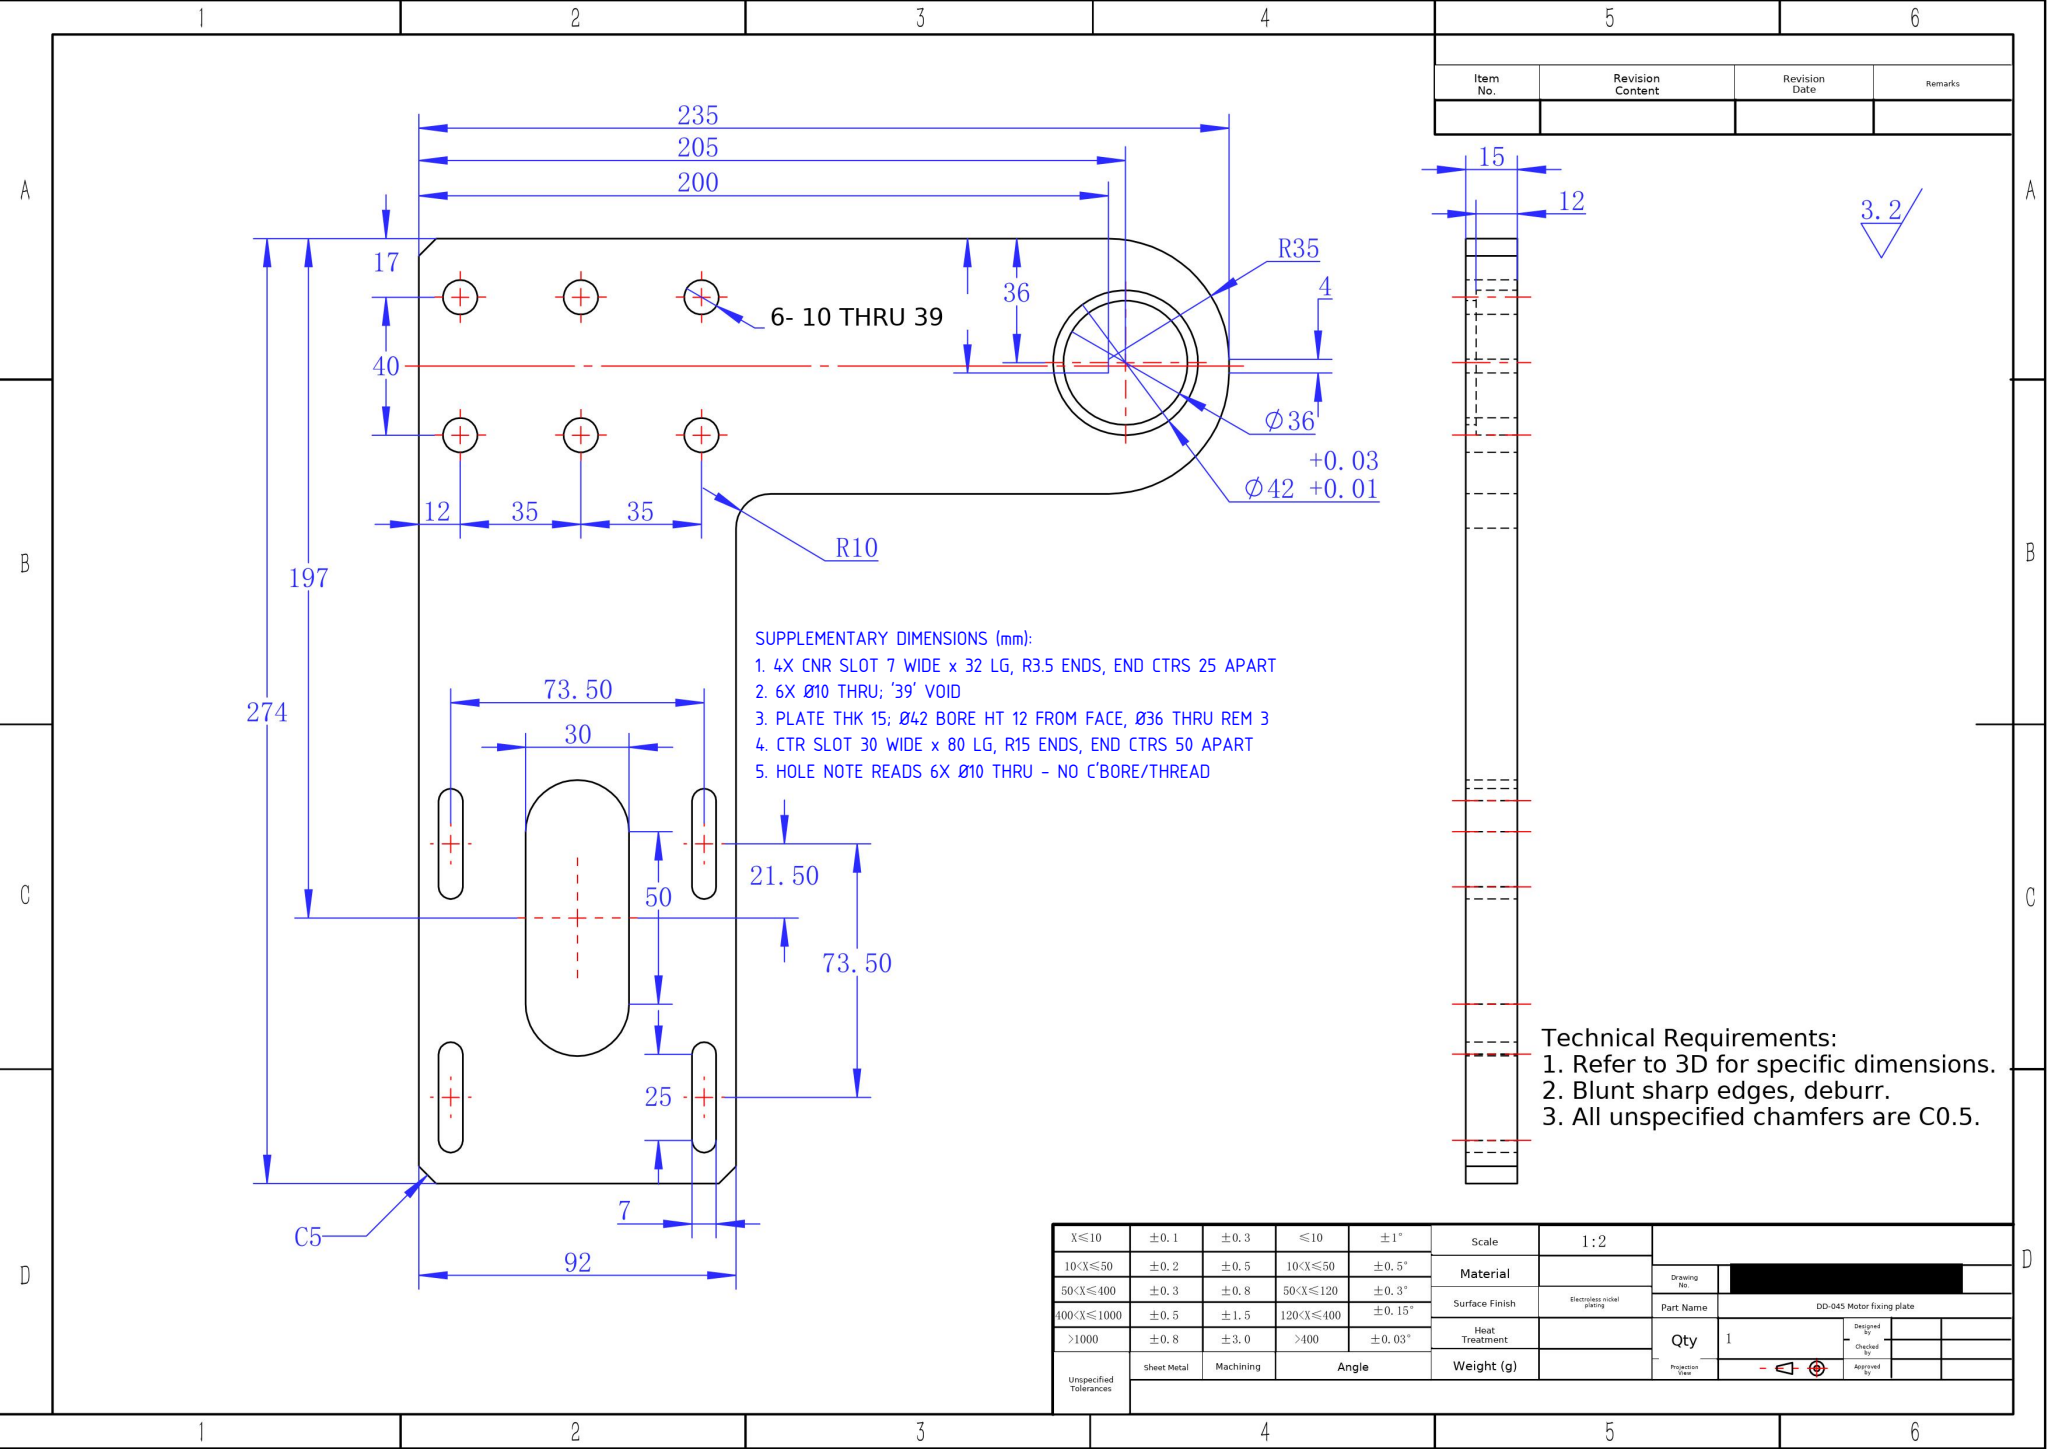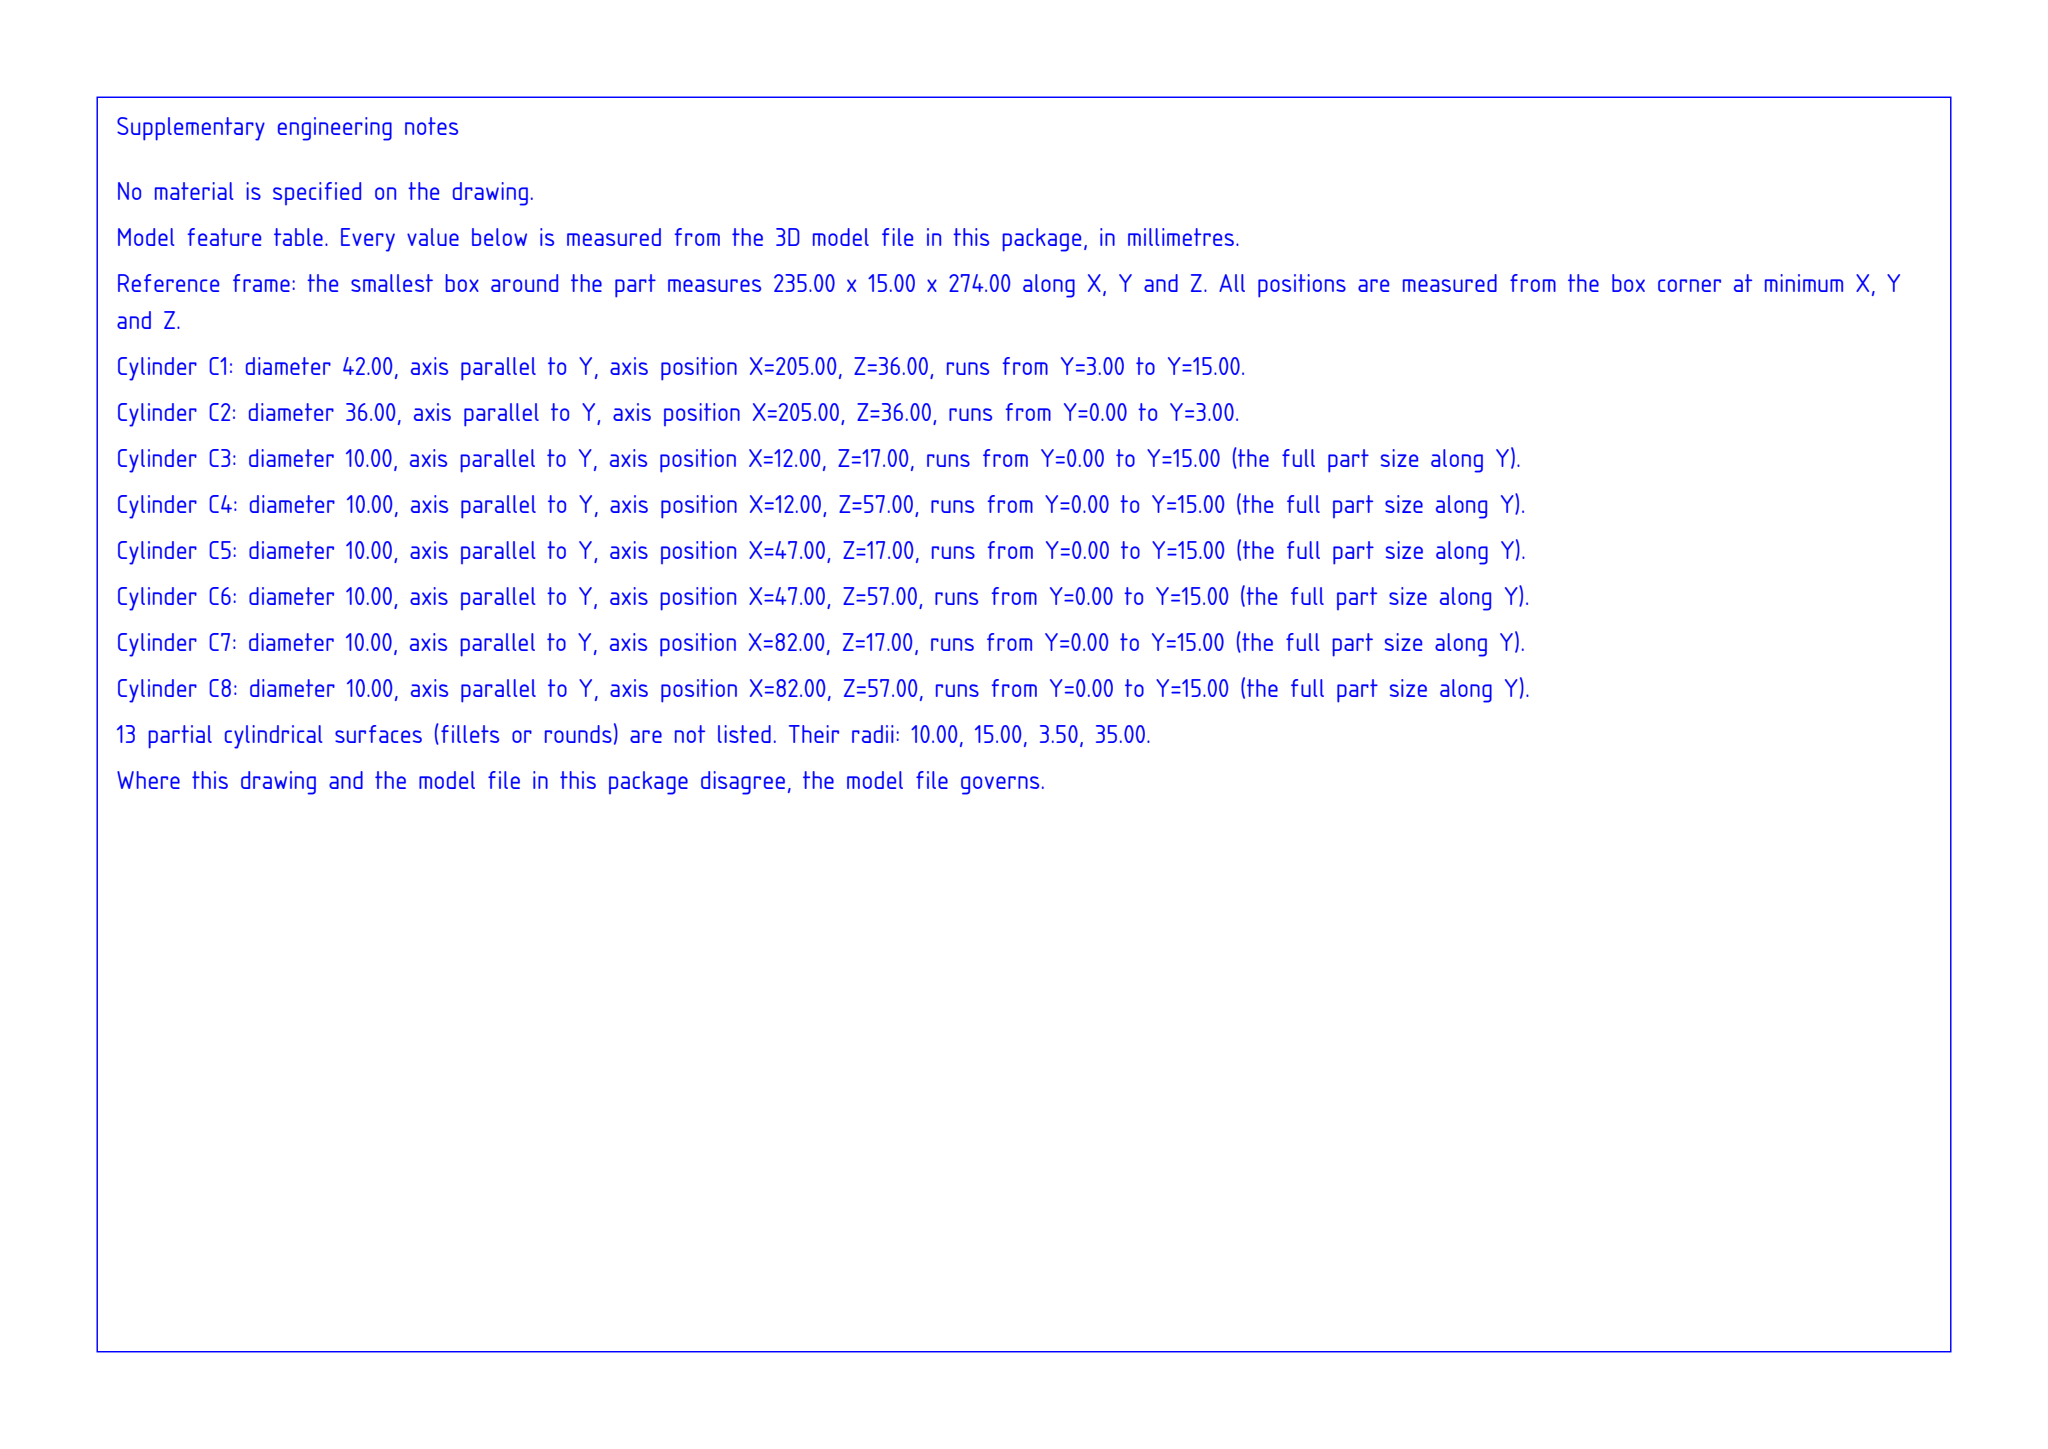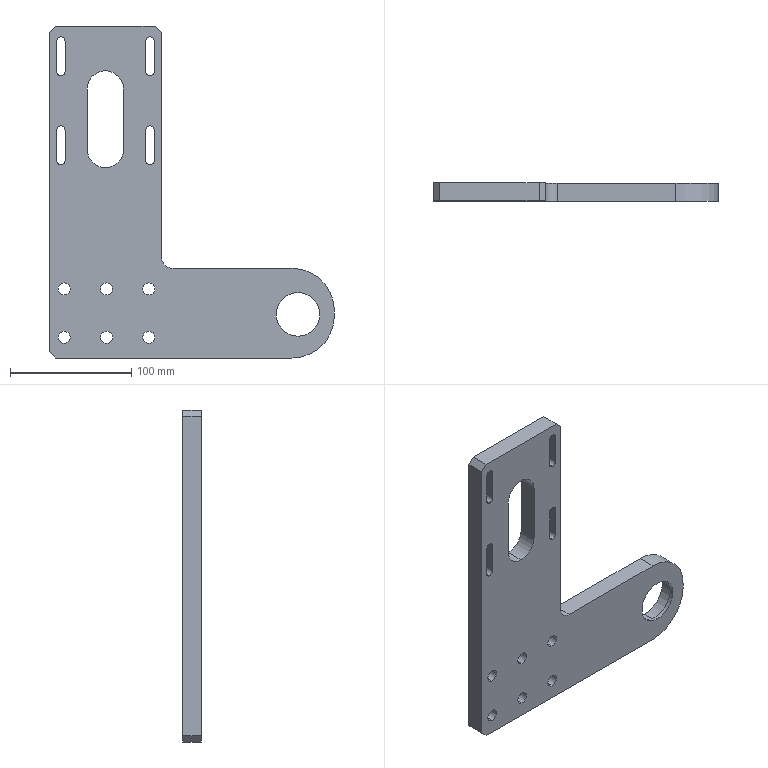Part | SolidWorks | mm | 1 solid | 56 faces | box 235 x 15 x 274 mm | volume 456063 mm3 | cylinder 34 | plane 22 | commonest cylinder face diameters 7 x12 10 x12 30 x3 36 x2 42 x2 70 x2 20 x1
build123d program:
from build123d import *

# Parameters (mm, degrees)
SKETCH1_W           = 235
SKETCH1_H           = 74
BOSS_EXTRUDE1_DEPTH = 15
SKETCH2_R           = 21
CUT_EXTRUDE1_DEPTH  = 12
SKETCH3_R           = 18
CUT_EXTRUDE2_DEPTH  = 124.771
SKETCH4_R           = 5
CUT_EXTRUDE3_DEPTH  = 125.098
FILLET1_R           = 35
SKETCH5_W           = 92
SKETCH5_H           = 15
BOSS_EXTRUDE2_DEPTH = 200
CUT_EXTRUDE4_DEPTH  = 265.953
CUT_EXTRUDE5_DEPTH  = 265.953
FILLET2_R           = 10
CHAMFER1_SIZE       = 5


with BuildPart() as part:
    # Sketch1 → Boss-Extrude1 (new body)
    with BuildSketch(Plane(origin=(0, 0, 0), x_dir=(1, 0, 0), z_dir=(0, 1, 0))):
        Rectangle(SKETCH1_W, SKETCH1_H)
    extrude(amount=BOSS_EXTRUDE1_DEPTH)

    # Sketch2 → Cut-Extrude1 (cut)
    with BuildSketch(Plane(origin=(0, 15, 0), x_dir=(1, 0, 0), z_dir=(0, 1, 0))):
        with Locations(Location((87.5, 1, 0), (0, 0, 270))):
            Circle(SKETCH2_R)
    extrude(amount=-CUT_EXTRUDE1_DEPTH, mode=Mode.SUBTRACT)

    # Sketch3 → Cut-Extrude2 (cut, through all)
    with BuildSketch(Plane(origin=(0, 3, 0), x_dir=(1, 0, 0), z_dir=(0, 1, 0))):
        with Locations(Location((87.5, 1, 0), (0, 0, 270))):
            Circle(SKETCH3_R)
    extrude(amount=-CUT_EXTRUDE2_DEPTH, mode=Mode.SUBTRACT)

    # Sketch4 → Cut-Extrude3 (cut, through all)
    with BuildSketch(Plane.XZ):
        with Locations(Location((-105.5, 20, 0), (0, 0, 270))):
            Circle(SKETCH4_R)
        with Locations(Location((-70.5, 20, 0), (0, 0, 270))):
            Circle(SKETCH4_R)
        with Locations(Location((-35.5, 20, 0), (0, 0, 270))):
            Circle(SKETCH4_R)
        with Locations(Location((-105.5, -20, 0), (0, 0, 270))):
            Circle(SKETCH4_R)
        with Locations(Location((-70.5, -20, 0), (0, 0, 270))):
            Circle(SKETCH4_R)
        with Locations(Location((-35.5, -20, 0), (0, 0, 270))):
            Circle(SKETCH4_R)
    extrude(amount=-CUT_EXTRUDE3_DEPTH, mode=Mode.SUBTRACT)

    # Fillet1
    fillet1_edges = [part.edges().sort_by_distance(p)[0] for p in [
        (117.5, 7.5, -37),
        (117.5, 7.5, 37),
    ]]
    fillet(fillet1_edges, radius=FILLET1_R)

    # Sketch5 → Boss-Extrude2 (add)
    with BuildSketch(Plane.XY.offset(37)):
        with Locations((-71.5, 7.5)):
            Rectangle(SKETCH5_W, SKETCH5_H)
    extrude(amount=BOSS_EXTRUDE2_DEPTH)

    # Sketch6 → Cut-Extrude4 (cut, through all)
    with BuildSketch(Plane.XZ):
        with BuildLine():
            Line((-38.25, 126), (-38.25, 151))
            ThreePointArc((-38.25, 151), (-34.75, 154.5), (-31.25, 151))
            Line((-31.25, 151), (-31.25, 126))
            ThreePointArc((-31.25, 126), (-34.75, 122.5), (-38.25, 126))
        make_face()
        with BuildLine():
            Line((-111.75, 126), (-111.75, 151))
            ThreePointArc((-111.75, 151), (-108.25, 154.5), (-104.75, 151))
            Line((-104.75, 151), (-104.75, 126))
            ThreePointArc((-104.75, 126), (-108.25, 122.5), (-111.75, 126))
        make_face()
        with BuildLine():
            Line((-38.25, 199.5), (-38.25, 224.5))
            ThreePointArc((-38.25, 224.5), (-34.75, 228), (-31.25, 224.5))
            Line((-31.25, 224.5), (-31.25, 199.5))
            ThreePointArc((-31.25, 199.5), (-34.75, 196), (-38.25, 199.5))
        make_face()
        with BuildLine():
            Line((-111.75, 199.5), (-111.75, 224.5))
            ThreePointArc((-111.75, 224.5), (-108.25, 228), (-104.75, 224.5))
            Line((-104.75, 224.5), (-104.75, 199.5))
            ThreePointArc((-104.75, 199.5), (-108.25, 196), (-111.75, 199.5))
        make_face()
    extrude(amount=-CUT_EXTRUDE4_DEPTH, mode=Mode.SUBTRACT)

    # Sketch7 → Cut-Extrude5 (cut, through all)
    with BuildSketch(Plane.XZ):
        with BuildLine():
            Line((-86.5, 135), (-86.5, 185))
            ThreePointArc((-86.5, 185), (-71.5, 200), (-56.5, 185))
            Line((-56.5, 185), (-56.5, 135))
            ThreePointArc((-56.5, 135), (-71.5, 120), (-86.5, 135))
        make_face()
    extrude(amount=-CUT_EXTRUDE5_DEPTH, mode=Mode.SUBTRACT)

    # Fillet2
    fillet2_edges = [part.edges().sort_by_distance(p)[0] for p in [
        (-25.5, 7.5, 37),
    ]]
    fillet(fillet2_edges, radius=FILLET2_R)

    # Chamfer1
    chamfer1_edges = [part.edges().sort_by_distance(p)[0] for p in [
        (-117.5, 7.5, 237),
        (-25.5, 7.5, 237),
        (-117.5, 7.5, -37),
    ]]
    chamfer(chamfer1_edges, length=CHAMFER1_SIZE)


solid = part.part